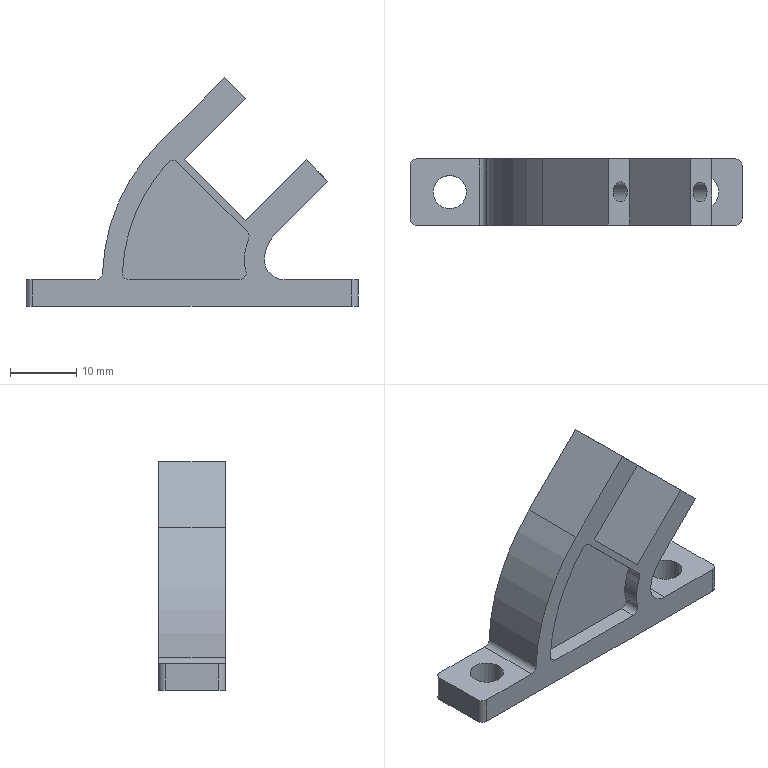Component | NX | INCLINED_FRAME | 1 solid | 48 faces | volume 5111 mm3 | cylinder 26 | plane 22 | commonest cylinder face diameters 2 x13 5 x2 3 x2 52 x2 12 x2 18.315 x2 58 x1 12.315 x1